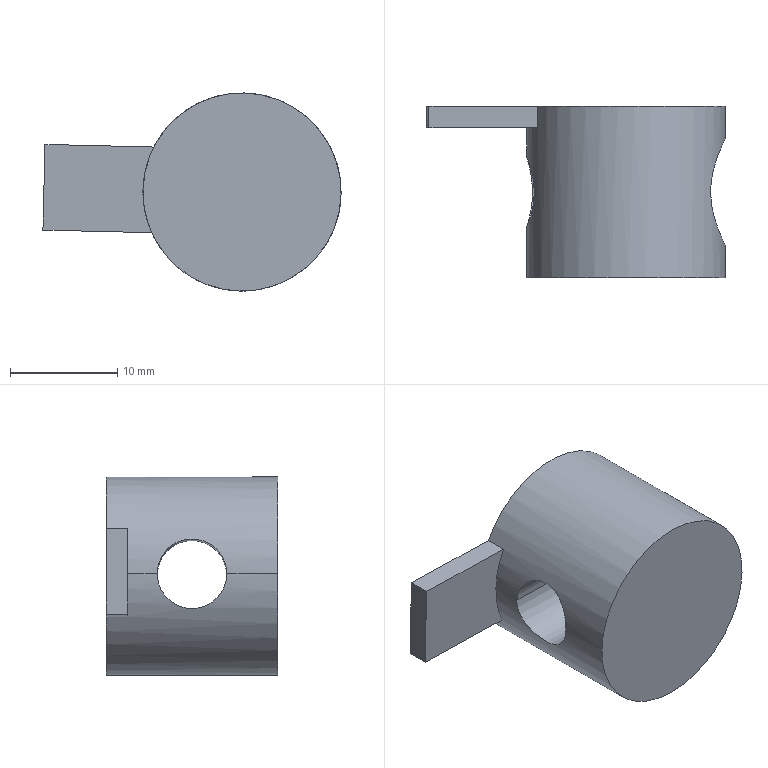Component | SolidWorks | 2012MB0201-1_AUpperRackFrameModule-1_ADJ42-G408-D6.5Assembly-10_Built-inConnectorADJ42-G408-D6.5-1 | 1 solid | 13 faces | box 27.84 x 16 x 18.5 mm | volume 3328 mm3 | plane 7 | cylinder 6 | commonest cylinder face diameters 10 x2 6.5 x2 18.5 x2 | material S45C
build123d program:
from build123d import *

# Parameters (mm, degrees)
SKETCH1_W                                     = 16
SKETCH1_H                                     = 9.25
COUNTERBORE_FOR_M6_HEX_HEAD_BOLT1_D           = 6.5
COUNTERBORE_FOR_M6_HEX_HEAD_BOLT1_CBORE_D     = 10
COUNTERBORE_FOR_M6_HEX_HEAD_BOLT1_CBORE_DEPTH = 12
BOSS_EXTRUDE1_REACH                           = 35.341
BOSS_EXTRUDE1_END_RADIUS                      = 9.25
SKETCH4_W                                     = 2
SKETCH4_H                                     = 8


with BuildPart() as part:
    # Sketch1 → Revolve1 (revolve)
    with BuildSketch(Plane.XY.offset(-18.5), mode=Mode.PRIVATE) as revolve1_sk:
        with Locations((8, 4.625)):
            Rectangle(SKETCH1_W, SKETCH1_H)
    revolve(revolve1_sk.sketch.rotate(Axis((0, 0, -18.5), (1, 0, 0)), 270), axis=Axis((0, 0, -18.5), (1, 0, 0)))

    # Counterbore for M6 Hex Head Bolt1 (through all)
    with Locations(Plane(origin=(8, 0, -27.75), x_dir=(-1, 0, 0), z_dir=(0, 0, -1))):
        with Locations((0, 0)):
            CounterBoreHole(COUNTERBORE_FOR_M6_HEX_HEAD_BOLT1_D / 2, COUNTERBORE_FOR_M6_HEX_HEAD_BOLT1_CBORE_D / 2, COUNTERBORE_FOR_M6_HEX_HEAD_BOLT1_CBORE_DEPTH)

    # Boss-Extrude1: up to this cylinder (the profile starts outside it)
    boss_extrude1_end = Plane(origin=(1, 0, -18.5), z_dir=(1, 0, 0)) * Cylinder(BOSS_EXTRUDE1_END_RADIUS, 90.182, mode=Mode.PRIVATE)
    # Sketch4 → Boss-Extrude1 (add, up to the surface)
    with BuildSketch(Plane.XY, mode=Mode.PRIVATE) as boss_extrude1_sk1:
        with Locations((1, 0)):
            Rectangle(SKETCH4_W, SKETCH4_H)
    boss_extrude1_tool1 = extrude(boss_extrude1_sk1.sketch, amount=-BOSS_EXTRUDE1_REACH, mode=Mode.PRIVATE) - boss_extrude1_end
    add(boss_extrude1_tool1.solids().sort_by_distance((1, 0, 0))[0])


solid = part.part

# Placed as in the assembly
solid = solid.moved(Location((-1764.43, 1041.85, -1140.078), (-0.007146, -88.631, -90.007)))
STEP:
#1=COLOUR_RGB('',0.7922,0.8196,0.9333);
#2=FILL_AREA_STYLE_COLOUR('',#1);
#3=FILL_AREA_STYLE('',(#2));
#4=SURFACE_STYLE_FILL_AREA(#3);
#5=SURFACE_SIDE_STYLE('',(#4));
#6=SURFACE_STYLE_USAGE(.BOTH.,#5);
#7=PRESENTATION_STYLE_ASSIGNMENT((#6));
#8=CARTESIAN_POINT('',(-68.846,40.506,-44.9));
#9=VERTEX_POINT('',#8);
#10=CARTESIAN_POINT('',(-68.846,40.9,-44.9));
#11=VERTEX_POINT('',#10);
#12=CARTESIAN_POINT('',(-68.846,40.703,-44.9));
#13=DIRECTION('',(0.9997,0.,-0.02392));
#14=DIRECTION('',(0.,1.,0.));
#15=AXIS2_PLACEMENT_3D('',#12,#13,#14);
#16=CIRCLE('',#15,0.1969);
#17=EDGE_CURVE('',#9,#11,#16,.T.);
#18=ORIENTED_EDGE('',*,*,#17,.F.);
#19=CARTESIAN_POINT('',(-68.374,40.506,-44.911));
#20=VERTEX_POINT('',#19);
#21=CARTESIAN_POINT('',(-68.374,40.506,-44.911));
#22=DIRECTION('',(0.9997,0.,-0.02392));
#23=VECTOR('',#22,39.37);
#24=LINE('',#21,#23);
#25=EDGE_CURVE('',#9,#20,#24,.T.);
#26=ORIENTED_EDGE('',*,*,#25,.T.);
#27=CARTESIAN_POINT('',(-68.374,40.9,-44.911));
#28=VERTEX_POINT('',#27);
#29=CARTESIAN_POINT('',(-68.374,40.506,-44.911));
#30=CARTESIAN_POINT('',(-68.374,40.506,-44.924));
#31=CARTESIAN_POINT('',(-68.375,40.507,-44.937));
#32=CARTESIAN_POINT('',(-68.378,40.512,-44.963));
#33=CARTESIAN_POINT('',(-68.381,40.516,-44.975));
#34=CARTESIAN_POINT('',(-68.386,40.526,-44.999));
#35=CARTESIAN_POINT('',(-68.39,40.532,-45.01));
#36=CARTESIAN_POINT('',(-68.397,40.547,-45.031));
#37=CARTESIAN_POINT('',(-68.401,40.555,-45.041));
#38=CARTESIAN_POINT('',(-68.409,40.573,-45.059));
#39=CARTESIAN_POINT('',(-68.412,40.582,-45.066));
#40=CARTESIAN_POINT('',(-68.42,40.604,-45.08));
#41=CARTESIAN_POINT('',(-68.423,40.615,-45.086));
#42=CARTESIAN_POINT('',(-68.429,40.638,-45.096));
#43=CARTESIAN_POINT('',(-68.432,40.651,-45.1));
#44=CARTESIAN_POINT('',(-68.435,40.676,-45.105));
#45=CARTESIAN_POINT('',(-68.436,40.689,-45.106));
#46=CARTESIAN_POINT('',(-68.436,40.716,-45.106));
#47=CARTESIAN_POINT('',(-68.435,40.729,-45.105));
#48=CARTESIAN_POINT('',(-68.432,40.754,-45.1));
#49=CARTESIAN_POINT('',(-68.429,40.767,-45.096));
#50=CARTESIAN_POINT('',(-68.423,40.791,-45.087));
#51=CARTESIAN_POINT('',(-68.42,40.802,-45.081));
#52=CARTESIAN_POINT('',(-68.412,40.823,-45.067));
#53=CARTESIAN_POINT('',(-68.409,40.833,-45.059));
#54=CARTESIAN_POINT('',(-68.401,40.851,-45.041));
#55=CARTESIAN_POINT('',(-68.397,40.859,-45.031));
#56=CARTESIAN_POINT('',(-68.391,40.869,-45.016));
#57=CARTESIAN_POINT('',(-68.39,40.873,-45.01));
#58=CARTESIAN_POINT('',(-68.386,40.879,-44.999));
#59=CARTESIAN_POINT('',(-68.385,40.882,-44.993));
#60=CARTESIAN_POINT('',(-68.381,40.889,-44.976));
#61=CARTESIAN_POINT('',(-68.378,40.893,-44.963));
#62=CARTESIAN_POINT('',(-68.375,40.898,-44.938));
#63=CARTESIAN_POINT('',(-68.374,40.9,-44.924));
#64=CARTESIAN_POINT('',(-68.374,40.9,-44.911));
#65=B_SPLINE_CURVE_WITH_KNOTS('',3,(#29,#30,#31,#32,#33,#34,#35,#36,#37,#38,#39,#40,#41,#42,#43,#44,#45,#46,#47,#48,#49,#50,#51,#52,#53,#54,#55,#56,#57,#58,#59,#60,#61,#62,#63,#64),.UNSPECIFIED.,.F.,.F.,(4,2,2,2,2,2,2,2,2,2,2,2,2,2,2,2,2,4),(0.01596,0.01695,0.01795,0.01894,0.01994,0.02093,0.02193,0.02292,0.02392,0.02491,0.02591,0.0269,0.0279,0.02889,0.02939,0.02989,0.03088,0.03188),.UNSPECIFIED.);
#66=EDGE_CURVE('',#20,#28,#65,.T.);
#67=ORIENTED_EDGE('',*,*,#66,.T.);
#68=CARTESIAN_POINT('',(-68.374,40.9,-44.911));
#69=DIRECTION('',(0.9997,0.,-0.02392));
#70=VECTOR('',#69,39.37);
#71=LINE('',#68,#70);
#72=EDGE_CURVE('',#11,#28,#71,.T.);
#73=ORIENTED_EDGE('',*,*,#72,.F.);
#74=EDGE_LOOP('',(#18,#26,#67,#73));
#75=FACE_OUTER_BOUND('',#74,.T.);
#76=CARTESIAN_POINT('',(-68.374,40.703,-44.911));
#77=DIRECTION('',(0.9997,0.,-0.02392));
#78=DIRECTION('',(0.,1.,0.));
#79=AXIS2_PLACEMENT_3D('',#76,#77,#78);
#80=CYLINDRICAL_SURFACE('',#79,0.1969);
#81=ADVANCED_FACE('',(#75),#80,.F.);
#82=CARTESIAN_POINT('',(-69.102,40.831,-44.894));
#83=VERTEX_POINT('',#82);
#84=CARTESIAN_POINT('',(-69.102,40.575,-44.894));
#85=VERTEX_POINT('',#84);
#86=CARTESIAN_POINT('',(-69.102,40.831,-44.894));
#87=CARTESIAN_POINT('',(-69.102,40.831,-44.902));
#88=CARTESIAN_POINT('',(-69.102,40.83,-44.911));
#89=CARTESIAN_POINT('',(-69.101,40.827,-44.927));
#90=CARTESIAN_POINT('',(-69.1,40.824,-44.935));
#91=CARTESIAN_POINT('',(-69.099,40.818,-44.951));
#92=CARTESIAN_POINT('',(-69.098,40.814,-44.958));
#93=CARTESIAN_POINT('',(-69.095,40.804,-44.972));
#94=CARTESIAN_POINT('',(-69.094,40.799,-44.979));
#95=CARTESIAN_POINT('',(-69.09,40.781,-44.996));
#96=CARTESIAN_POINT('',(-69.087,40.767,-45.006));
#97=CARTESIAN_POINT('',(-69.084,40.744,-45.015));
#98=CARTESIAN_POINT('',(-69.083,40.736,-45.018));
#99=CARTESIAN_POINT('',(-69.082,40.72,-45.021));
#100=CARTESIAN_POINT('',(-69.082,40.711,-45.022));
#101=CARTESIAN_POINT('',(-69.082,40.694,-45.022));
#102=CARTESIAN_POINT('',(-69.082,40.686,-45.021));
#103=CARTESIAN_POINT('',(-69.083,40.669,-45.018));
#104=CARTESIAN_POINT('',(-69.084,40.661,-45.015));
#105=CARTESIAN_POINT('',(-69.086,40.646,-45.009));
#106=CARTESIAN_POINT('',(-69.087,40.638,-45.005));
#107=CARTESIAN_POINT('',(-69.09,40.625,-44.996));
#108=CARTESIAN_POINT('',(-69.091,40.618,-44.99));
#109=CARTESIAN_POINT('',(-69.094,40.606,-44.978));
#110=CARTESIAN_POINT('',(-69.095,40.601,-44.972));
#111=CARTESIAN_POINT('',(-69.098,40.592,-44.958));
#112=CARTESIAN_POINT('',(-69.099,40.588,-44.951));
#113=CARTESIAN_POINT('',(-69.1,40.581,-44.935));
#114=CARTESIAN_POINT('',(-69.101,40.579,-44.927));
#115=CARTESIAN_POINT('',(-69.102,40.576,-44.911));
#116=CARTESIAN_POINT('',(-69.102,40.575,-44.902));
#117=CARTESIAN_POINT('',(-69.102,40.575,-44.894));
#118=B_SPLINE_CURVE_WITH_KNOTS('',3,(#86,#87,#88,#89,#90,#91,#92,#93,#94,#95,#96,#97,#98,#99,#100,#101,#102,#103,#104,#105,#106,#107,#108,#109,#110,#111,#112,#113,#114,#115,#116,#117),.UNSPECIFIED.,.F.,.F.,(4,2,2,2,2,2,2,2,2,2,2,2,2,2,2,4),(0.,0.0006402,0.00128,0.001921,0.002561,0.003841,0.004481,0.005122,0.005762,0.006402,0.007042,0.007683,0.008323,0.008963,0.009603,0.01024),.UNSPECIFIED.);
#119=EDGE_CURVE('',#83,#85,#118,.T.);
#120=ORIENTED_EDGE('',*,*,#119,.T.);
#121=CARTESIAN_POINT('',(-68.846,40.575,-44.9));
#122=VERTEX_POINT('',#121);
#123=CARTESIAN_POINT('',(-68.374,40.575,-44.911));
#124=DIRECTION('',(0.9997,0.,-0.02392));
#125=VECTOR('',#124,39.37);
#126=LINE('',#123,#125);
#127=EDGE_CURVE('',#85,#122,#126,.T.);
#128=ORIENTED_EDGE('',*,*,#127,.T.);
#129=CARTESIAN_POINT('',(-68.846,40.831,-44.9));
#130=VERTEX_POINT('',#129);
#131=CARTESIAN_POINT('',(-68.846,40.703,-44.9));
#132=DIRECTION('',(0.9997,0.,-0.02392));
#133=DIRECTION('',(0.,1.,0.));
#134=AXIS2_PLACEMENT_3D('',#131,#132,#133);
#135=CIRCLE('',#134,0.128);
#136=EDGE_CURVE('',#122,#130,#135,.T.);
#137=ORIENTED_EDGE('',*,*,#136,.T.);
#138=CARTESIAN_POINT('',(-68.374,40.831,-44.911));
#139=DIRECTION('',(0.9997,0.,-0.02392));
#140=VECTOR('',#139,39.37);
#141=LINE('',#138,#140);
#142=EDGE_CURVE('',#83,#130,#141,.T.);
#143=ORIENTED_EDGE('',*,*,#142,.F.);
#144=EDGE_LOOP('',(#120,#128,#137,#143));
#145=FACE_OUTER_BOUND('',#144,.T.);
#146=CARTESIAN_POINT('',(-68.374,40.703,-44.911));
#147=DIRECTION('',(0.9997,0.,-0.02392));
#148=DIRECTION('',(0.,1.,0.));
#149=AXIS2_PLACEMENT_3D('',#146,#147,#148);
#150=CYLINDRICAL_SURFACE('',#149,0.128);
#151=ADVANCED_FACE('',(#145),#150,.F.);
#152=CARTESIAN_POINT('',(-69.062,40.939,-44.737));
#153=VERTEX_POINT('',#152);
#154=CARTESIAN_POINT('',(-69.102,40.939,-44.894));
#155=VERTEX_POINT('',#154);
#156=CARTESIAN_POINT('',(-68.738,40.939,-44.902));
#157=DIRECTION('',(0.,-1.,-0.));
#158=DIRECTION('',(0.9997,0.,-0.02392));
#159=AXIS2_PLACEMENT_3D('',#156,#157,#158);
#160=CIRCLE('',#159,0.3642);
#161=EDGE_CURVE('',#153,#155,#160,.T.);
#162=ORIENTED_EDGE('',*,*,#161,.T.);
#163=CARTESIAN_POINT('',(-69.102,41.018,-44.894));
#164=DIRECTION('',(0.,-1.,-0.));
#165=VECTOR('',#164,39.37);
#166=LINE('',#163,#165);
#167=EDGE_CURVE('',#155,#83,#166,.T.);
#168=ORIENTED_EDGE('',*,*,#167,.T.);
#169=CARTESIAN_POINT('',(-69.102,40.575,-44.894));
#170=CARTESIAN_POINT('',(-69.101,40.575,-44.885));
#171=CARTESIAN_POINT('',(-69.101,40.576,-44.877));
#172=CARTESIAN_POINT('',(-69.099,40.579,-44.86));
#173=CARTESIAN_POINT('',(-69.098,40.581,-44.852));
#174=CARTESIAN_POINT('',(-69.096,40.588,-44.837));
#175=CARTESIAN_POINT('',(-69.094,40.592,-44.829));
#176=CARTESIAN_POINT('',(-69.091,40.601,-44.816));
#177=CARTESIAN_POINT('',(-69.09,40.606,-44.809));
#178=CARTESIAN_POINT('',(-69.086,40.618,-44.798));
#179=CARTESIAN_POINT('',(-69.085,40.625,-44.792));
#180=CARTESIAN_POINT('',(-69.082,40.638,-44.783));
#181=CARTESIAN_POINT('',(-69.08,40.646,-44.779));
#182=CARTESIAN_POINT('',(-69.078,40.661,-44.773));
#183=CARTESIAN_POINT('',(-69.077,40.669,-44.77));
#184=CARTESIAN_POINT('',(-69.076,40.686,-44.767));
#185=CARTESIAN_POINT('',(-69.075,40.694,-44.766));
#186=CARTESIAN_POINT('',(-69.075,40.711,-44.766));
#187=CARTESIAN_POINT('',(-69.076,40.72,-44.767));
#188=CARTESIAN_POINT('',(-69.077,40.736,-44.77));
#189=CARTESIAN_POINT('',(-69.078,40.744,-44.773));
#190=CARTESIAN_POINT('',(-69.08,40.76,-44.779));
#191=CARTESIAN_POINT('',(-69.082,40.767,-44.783));
#192=CARTESIAN_POINT('',(-69.085,40.781,-44.792));
#193=CARTESIAN_POINT('',(-69.086,40.787,-44.798));
#194=CARTESIAN_POINT('',(-69.09,40.799,-44.809));
#195=CARTESIAN_POINT('',(-69.091,40.804,-44.816));
#196=CARTESIAN_POINT('',(-69.094,40.814,-44.83));
#197=CARTESIAN_POINT('',(-69.096,40.818,-44.837));
#198=CARTESIAN_POINT('',(-69.098,40.824,-44.852));
#199=CARTESIAN_POINT('',(-69.099,40.827,-44.86));
#200=CARTESIAN_POINT('',(-69.101,40.83,-44.877));
#201=CARTESIAN_POINT('',(-69.101,40.831,-44.885));
#202=CARTESIAN_POINT('',(-69.102,40.831,-44.894));
#203=B_SPLINE_CURVE_WITH_KNOTS('',3,(#169,#170,#171,#172,#173,#174,#175,#176,#177,#178,#179,#180,#181,#182,#183,#184,#185,#186,#187,#188,#189,#190,#191,#192,#193,#194,#195,#196,#197,#198,#199,#200,#201,#202),.UNSPECIFIED.,.F.,.F.,(4,2,2,2,2,2,2,2,2,2,2,2,2,2,2,2,4),(0.01024,0.01088,0.01152,0.01216,0.0128,0.01344,0.01408,0.01472,0.01536,0.016,0.01664,0.01728,0.01792,0.01856,0.0192,0.01984,0.02048),.UNSPECIFIED.);
#204=EDGE_CURVE('',#85,#83,#203,.T.);
#205=ORIENTED_EDGE('',*,*,#204,.F.);
#206=CARTESIAN_POINT('',(-69.102,40.388,-44.894));
#207=VERTEX_POINT('',#206);
#208=CARTESIAN_POINT('',(-69.102,41.018,-44.894));
#209=DIRECTION('',(0.,-1.,-0.));
#210=VECTOR('',#209,39.37);
#211=LINE('',#208,#210);
#212=EDGE_CURVE('',#85,#207,#211,.T.);
#213=ORIENTED_EDGE('',*,*,#212,.T.);
#214=CARTESIAN_POINT('',(-68.374,40.388,-44.911));
#215=VERTEX_POINT('',#214);
#216=CARTESIAN_POINT('',(-68.738,40.388,-44.902));
#217=DIRECTION('',(0.,-1.,-0.));
#218=DIRECTION('',(0.9997,0.,-0.02392));
#219=AXIS2_PLACEMENT_3D('',#216,#217,#218);
#220=CIRCLE('',#219,0.3642);
#221=EDGE_CURVE('',#215,#207,#220,.T.);
#222=ORIENTED_EDGE('',*,*,#221,.F.);
#223=CARTESIAN_POINT('',(-68.374,41.018,-44.911));
#224=DIRECTION('',(0.,-1.,-0.));
#225=VECTOR('',#224,39.37);
#226=LINE('',#223,#225);
#227=EDGE_CURVE('',#20,#215,#226,.T.);
#228=ORIENTED_EDGE('',*,*,#227,.F.);
#229=CARTESIAN_POINT('',(-68.374,40.9,-44.911));
#230=CARTESIAN_POINT('',(-68.373,40.9,-44.898));
#231=CARTESIAN_POINT('',(-68.374,40.898,-44.885));
#232=CARTESIAN_POINT('',(-68.376,40.893,-44.859));
#233=CARTESIAN_POINT('',(-68.378,40.889,-44.846));
#234=CARTESIAN_POINT('',(-68.382,40.879,-44.823));
#235=CARTESIAN_POINT('',(-68.385,40.873,-44.811));
#236=CARTESIAN_POINT('',(-68.391,40.859,-44.79));
#237=CARTESIAN_POINT('',(-68.394,40.851,-44.78));
#238=CARTESIAN_POINT('',(-68.401,40.833,-44.762));
#239=CARTESIAN_POINT('',(-68.405,40.823,-44.754));
#240=CARTESIAN_POINT('',(-68.412,40.802,-44.74));
#241=CARTESIAN_POINT('',(-68.415,40.791,-44.733));
#242=CARTESIAN_POINT('',(-68.42,40.767,-44.723));
#243=CARTESIAN_POINT('',(-68.423,40.755,-44.719));
#244=CARTESIAN_POINT('',(-68.426,40.729,-44.714));
#245=CARTESIAN_POINT('',(-68.427,40.716,-44.713));
#246=CARTESIAN_POINT('',(-68.427,40.696,-44.713));
#247=CARTESIAN_POINT('',(-68.426,40.69,-44.713));
#248=CARTESIAN_POINT('',(-68.426,40.677,-44.715));
#249=CARTESIAN_POINT('',(-68.425,40.67,-44.716));
#250=CARTESIAN_POINT('',(-68.423,40.657,-44.718));
#251=CARTESIAN_POINT('',(-68.423,40.651,-44.72));
#252=CARTESIAN_POINT('',(-68.42,40.639,-44.724));
#253=CARTESIAN_POINT('',(-68.419,40.633,-44.726));
#254=CARTESIAN_POINT('',(-68.415,40.615,-44.733));
#255=CARTESIAN_POINT('',(-68.412,40.604,-44.74));
#256=CARTESIAN_POINT('',(-68.405,40.582,-44.754));
#257=CARTESIAN_POINT('',(-68.401,40.573,-44.762));
#258=CARTESIAN_POINT('',(-68.394,40.555,-44.78));
#259=CARTESIAN_POINT('',(-68.391,40.547,-44.79));
#260=CARTESIAN_POINT('',(-68.385,40.532,-44.811));
#261=CARTESIAN_POINT('',(-68.382,40.526,-44.823));
#262=CARTESIAN_POINT('',(-68.379,40.519,-44.841));
#263=CARTESIAN_POINT('',(-68.378,40.517,-44.847));
#264=CARTESIAN_POINT('',(-68.376,40.513,-44.859));
#265=CARTESIAN_POINT('',(-68.375,40.511,-44.866));
#266=CARTESIAN_POINT('',(-68.374,40.507,-44.885));
#267=CARTESIAN_POINT('',(-68.373,40.506,-44.898));
#268=CARTESIAN_POINT('',(-68.374,40.506,-44.911));
#269=B_SPLINE_CURVE_WITH_KNOTS('',3,(#229,#230,#231,#232,#233,#234,#235,#236,#237,#238,#239,#240,#241,#242,#243,#244,#245,#246,#247,#248,#249,#250,#251,#252,#253,#254,#255,#256,#257,#258,#259,#260,#261,#262,#263,#264,#265,#266,#267,#268),.UNSPECIFIED.,.F.,.F.,(4,2,2,2,2,2,2,2,2,2,2,2,2,2,2,2,2,2,2,4),(0.,0.0009973,0.001995,0.002992,0.003989,0.004987,0.005984,0.006981,0.007979,0.008477,0.008976,0.009475,0.009973,0.01097,0.01197,0.01297,0.01396,0.01446,0.01496,0.01596),.UNSPECIFIED.);
#270=EDGE_CURVE('',#28,#20,#269,.T.);
#271=ORIENTED_EDGE('',*,*,#270,.F.);
#272=CARTESIAN_POINT('',(-68.374,41.018,-44.911));
#273=VERTEX_POINT('',#272);
#274=CARTESIAN_POINT('',(-68.374,41.018,-44.911));
#275=DIRECTION('',(0.,-1.,-0.));
#276=VECTOR('',#275,39.37);
#277=LINE('',#274,#276);
#278=EDGE_CURVE('',#273,#28,#277,.T.);
#279=ORIENTED_EDGE('',*,*,#278,.F.);
#280=CARTESIAN_POINT('',(-69.062,41.018,-44.737));
#281=VERTEX_POINT('',#280);
#282=CARTESIAN_POINT('',(-68.738,41.018,-44.902));
#283=DIRECTION('',(0.,-1.,-0.));
#284=DIRECTION('',(0.9997,0.,-0.02392));
#285=AXIS2_PLACEMENT_3D('',#282,#283,#284);
#286=CIRCLE('',#285,0.3642);
#287=EDGE_CURVE('',#273,#281,#286,.T.);
#288=ORIENTED_EDGE('',*,*,#287,.T.);
#289=CARTESIAN_POINT('',(-69.062,41.018,-44.737));
#290=DIRECTION('',(0.,-1.,-0.));
#291=VECTOR('',#290,39.37);
#292=LINE('',#289,#291);
#293=EDGE_CURVE('',#281,#153,#292,.T.);
#294=ORIENTED_EDGE('',*,*,#293,.T.);
#295=EDGE_LOOP('',(#162,#168,#205,#213,#222,#228,#271,#279,#288,#294));
#296=FACE_OUTER_BOUND('',#295,.T.);
#297=CARTESIAN_POINT('',(-68.738,41.018,-44.902));
#298=DIRECTION('',(0.,-1.,-0.));
#299=DIRECTION('',(0.9997,0.,-0.02392));
#300=AXIS2_PLACEMENT_3D('',#297,#298,#299);
#301=CYLINDRICAL_SURFACE('',#300,0.3642);
#302=ADVANCED_FACE('',(#296),#301,.T.);
#303=ORIENTED_EDGE('',*,*,#167,.F.);
#304=CARTESIAN_POINT('',(-69.07,40.939,-45.052));
#305=VERTEX_POINT('',#304);
#306=CARTESIAN_POINT('',(-68.738,40.939,-44.902));
#307=DIRECTION('',(0.,-1.,-0.));
#308=DIRECTION('',(0.9997,0.,-0.02392));
#309=AXIS2_PLACEMENT_3D('',#306,#307,#308);
#310=CIRCLE('',#309,0.3642);
#311=EDGE_CURVE('',#155,#305,#310,.T.);
#312=ORIENTED_EDGE('',*,*,#311,.T.);
#313=CARTESIAN_POINT('',(-69.07,41.018,-45.052));
#314=VERTEX_POINT('',#313);
#315=CARTESIAN_POINT('',(-69.07,41.018,-45.052));
#316=DIRECTION('',(-0.,1.,0.));
#317=VECTOR('',#316,39.37);
#318=LINE('',#315,#317);
#319=EDGE_CURVE('',#305,#314,#318,.T.);
#320=ORIENTED_EDGE('',*,*,#319,.T.);
#321=CARTESIAN_POINT('',(-68.738,41.018,-44.902));
#322=DIRECTION('',(0.,-1.,-0.));
#323=DIRECTION('',(0.9997,0.,-0.02392));
#324=AXIS2_PLACEMENT_3D('',#321,#322,#323);
#325=CIRCLE('',#324,0.3642);
#326=EDGE_CURVE('',#314,#273,#325,.T.);
#327=ORIENTED_EDGE('',*,*,#326,.T.);
#328=ORIENTED_EDGE('',*,*,#278,.T.);
#329=ORIENTED_EDGE('',*,*,#66,.F.);
#330=ORIENTED_EDGE('',*,*,#227,.T.);
#331=CARTESIAN_POINT('',(-68.738,40.388,-44.902));
#332=DIRECTION('',(0.,-1.,-0.));
#333=DIRECTION('',(0.9997,0.,-0.02392));
#334=AXIS2_PLACEMENT_3D('',#331,#332,#333);
#335=CIRCLE('',#334,0.3642);
#336=EDGE_CURVE('',#207,#215,#335,.T.);
#337=ORIENTED_EDGE('',*,*,#336,.F.);
#338=ORIENTED_EDGE('',*,*,#212,.F.);
#339=ORIENTED_EDGE('',*,*,#119,.F.);
#340=EDGE_LOOP('',(#303,#312,#320,#327,#328,#329,#330,#337,#338,#339));
#341=FACE_OUTER_BOUND('',#340,.T.);
#342=CARTESIAN_POINT('',(-68.738,41.018,-44.902));
#343=DIRECTION('',(0.,-1.,-0.));
#344=DIRECTION('',(0.9997,0.,-0.02392));
#345=AXIS2_PLACEMENT_3D('',#342,#343,#344);
#346=CYLINDRICAL_SURFACE('',#345,0.3642);
#347=ADVANCED_FACE('',(#341),#346,.T.);
#348=ORIENTED_EDGE('',*,*,#326,.F.);
#349=CARTESIAN_POINT('',(-69.47,41.018,-45.042));
#350=VERTEX_POINT('',#349);
#351=CARTESIAN_POINT('',(-68.377,41.018,-45.068));
#352=DIRECTION('',(-0.9997,-0.,0.02392));
#353=VECTOR('',#352,39.37);
#354=LINE('',#351,#353);
#355=EDGE_CURVE('',#314,#350,#354,.T.);
#356=ORIENTED_EDGE('',*,*,#355,.T.);
#357=CARTESIAN_POINT('',(-69.462,41.018,-44.727));
#358=VERTEX_POINT('',#357);
#359=CARTESIAN_POINT('',(-69.462,41.018,-44.727));
#360=DIRECTION('',(-0.02392,0.,-0.9997));
#361=VECTOR('',#360,39.37);
#362=LINE('',#359,#361);
#363=EDGE_CURVE('',#358,#350,#362,.T.);
#364=ORIENTED_EDGE('',*,*,#363,.F.);
#365=CARTESIAN_POINT('',(-68.37,41.018,-44.754));
#366=DIRECTION('',(-0.9997,-0.,0.02392));
#367=VECTOR('',#366,39.37);
#368=LINE('',#365,#367);
#369=EDGE_CURVE('',#281,#358,#368,.T.);
#370=ORIENTED_EDGE('',*,*,#369,.F.);
#371=ORIENTED_EDGE('',*,*,#287,.F.);
#372=EDGE_LOOP('',(#348,#356,#364,#370,#371));
#373=FACE_OUTER_BOUND('',#372,.T.);
#374=CARTESIAN_POINT('',(-68.729,41.018,-44.538));
#375=DIRECTION('',(-0.,1.,0.));
#376=DIRECTION('',(-0.9997,-0.,0.02392));
#377=AXIS2_PLACEMENT_3D('',#374,#375,#376);
#378=PLANE('',#377);
#379=ADVANCED_FACE('',(#373),#378,.T.);
#380=ORIENTED_EDGE('',*,*,#221,.T.);
#381=ORIENTED_EDGE('',*,*,#336,.T.);
#382=EDGE_LOOP('',(#380,#381));
#383=FACE_OUTER_BOUND('',#382,.T.);
#384=CARTESIAN_POINT('',(-68.738,40.388,-44.902));
#385=DIRECTION('',(0.,-1.,-0.));
#386=DIRECTION('',(0.9997,0.,-0.02392));
#387=AXIS2_PLACEMENT_3D('',#384,#385,#386);
#388=PLANE('',#387);
#389=ADVANCED_FACE('',(#383),#388,.T.);
#390=ORIENTED_EDGE('',*,*,#127,.F.);
#391=ORIENTED_EDGE('',*,*,#204,.T.);
#392=ORIENTED_EDGE('',*,*,#142,.T.);
#393=CARTESIAN_POINT('',(-68.846,40.703,-44.9));
#394=DIRECTION('',(0.9997,0.,-0.02392));
#395=DIRECTION('',(0.,1.,0.));
#396=AXIS2_PLACEMENT_3D('',#393,#394,#395);
#397=CIRCLE('',#396,0.128);
#398=EDGE_CURVE('',#130,#122,#397,.T.);
#399=ORIENTED_EDGE('',*,*,#398,.T.);
#400=EDGE_LOOP('',(#390,#391,#392,#399));
#401=FACE_OUTER_BOUND('',#400,.T.);
#402=CARTESIAN_POINT('',(-68.374,40.703,-44.911));
#403=DIRECTION('',(0.9997,0.,-0.02392));
#404=DIRECTION('',(0.,1.,0.));
#405=AXIS2_PLACEMENT_3D('',#402,#403,#404);
#406=CYLINDRICAL_SURFACE('',#405,0.128);
#407=ADVANCED_FACE('',(#401),#406,.F.);
#408=ORIENTED_EDGE('',*,*,#398,.F.);
#409=ORIENTED_EDGE('',*,*,#136,.F.);
#410=EDGE_LOOP('',(#408,#409));
#411=FACE_BOUND('',#410,.T.);
#412=CARTESIAN_POINT('',(-68.846,40.703,-44.9));
#413=DIRECTION('',(0.9997,0.,-0.02392));
#414=DIRECTION('',(0.,1.,0.));
#415=AXIS2_PLACEMENT_3D('',#412,#413,#414);
#416=CIRCLE('',#415,0.1969);
#417=EDGE_CURVE('',#11,#9,#416,.T.);
#418=ORIENTED_EDGE('',*,*,#417,.T.);
#419=ORIENTED_EDGE('',*,*,#17,.T.);
#420=EDGE_LOOP('',(#418,#419));
#421=FACE_OUTER_BOUND('',#420,.T.);
#422=CARTESIAN_POINT('',(-68.846,40.575,-44.9));
#423=DIRECTION('',(-0.9997,-0.,0.02392));
#424=DIRECTION('',(0.,-1.,-0.));
#425=AXIS2_PLACEMENT_3D('',#422,#423,#424);
#426=PLANE('',#425);
#427=ADVANCED_FACE('',(#411,#421),#426,.F.);
#428=ORIENTED_EDGE('',*,*,#25,.F.);
#429=ORIENTED_EDGE('',*,*,#417,.F.);
#430=ORIENTED_EDGE('',*,*,#72,.T.);
#431=ORIENTED_EDGE('',*,*,#270,.T.);
#432=EDGE_LOOP('',(#428,#429,#430,#431));
#433=FACE_OUTER_BOUND('',#432,.T.);
#434=CARTESIAN_POINT('',(-68.374,40.703,-44.911));
#435=DIRECTION('',(0.9997,0.,-0.02392));
#436=DIRECTION('',(0.,1.,0.));
#437=AXIS2_PLACEMENT_3D('',#434,#435,#436);
#438=CYLINDRICAL_SURFACE('',#437,0.1969);
#439=ADVANCED_FACE('',(#433),#438,.F.);
#440=ORIENTED_EDGE('',*,*,#293,.F.);
#441=ORIENTED_EDGE('',*,*,#369,.T.);
#442=CARTESIAN_POINT('',(-69.462,40.939,-44.727));
#443=VERTEX_POINT('',#442);
#444=CARTESIAN_POINT('',(-69.462,40.939,-44.727));
#445=DIRECTION('',(-0.,1.,0.));
#446=VECTOR('',#445,39.37);
#447=LINE('',#444,#446);
#448=EDGE_CURVE('',#443,#358,#447,.T.);
#449=ORIENTED_EDGE('',*,*,#448,.F.);
#450=CARTESIAN_POINT('',(-68.37,40.939,-44.754));
#451=DIRECTION('',(-0.9997,-0.,0.02392));
#452=VECTOR('',#451,39.37);
#453=LINE('',#450,#452);
#454=EDGE_CURVE('',#153,#443,#453,.T.);
#455=ORIENTED_EDGE('',*,*,#454,.F.);
#456=EDGE_LOOP('',(#440,#441,#449,#455));
#457=FACE_OUTER_BOUND('',#456,.T.);
#458=CARTESIAN_POINT('',(-68.37,40.939,-44.754));
#459=DIRECTION('',(0.02392,-0.,0.9997));
#460=DIRECTION('',(-0.9997,-0.,0.02392));
#461=AXIS2_PLACEMENT_3D('',#458,#459,#460);
#462=PLANE('',#461);
#463=ADVANCED_FACE('',(#457),#462,.T.);
#464=ORIENTED_EDGE('',*,*,#363,.T.);
#465=CARTESIAN_POINT('',(-69.47,40.939,-45.042));
#466=VERTEX_POINT('',#465);
#467=CARTESIAN_POINT('',(-69.47,41.018,-45.042));
#468=DIRECTION('',(0.,-1.,-0.));
#469=VECTOR('',#468,39.37);
#470=LINE('',#467,#469);
#471=EDGE_CURVE('',#350,#466,#470,.T.);
#472=ORIENTED_EDGE('',*,*,#471,.T.);
#473=CARTESIAN_POINT('',(-69.47,40.939,-45.042));
#474=DIRECTION('',(0.02392,-0.,0.9997));
#475=VECTOR('',#474,39.37);
#476=LINE('',#473,#475);
#477=EDGE_CURVE('',#466,#443,#476,.T.);
#478=ORIENTED_EDGE('',*,*,#477,.T.);
#479=ORIENTED_EDGE('',*,*,#448,.T.);
#480=EDGE_LOOP('',(#464,#472,#478,#479));
#481=FACE_OUTER_BOUND('',#480,.T.);
#482=CARTESIAN_POINT('',(-69.466,41.018,-44.885));
#483=DIRECTION('',(-0.9997,-0.,0.02392));
#484=DIRECTION('',(0.,-1.,-0.));
#485=AXIS2_PLACEMENT_3D('',#482,#483,#484);
#486=PLANE('',#485);
#487=ADVANCED_FACE('',(#481),#486,.T.);
#488=ORIENTED_EDGE('',*,*,#161,.F.);
#489=ORIENTED_EDGE('',*,*,#454,.T.);
#490=ORIENTED_EDGE('',*,*,#477,.F.);
#491=CARTESIAN_POINT('',(-68.377,40.939,-45.068));
#492=DIRECTION('',(-0.9997,-0.,0.02392));
#493=VECTOR('',#492,39.37);
#494=LINE('',#491,#493);
#495=EDGE_CURVE('',#305,#466,#494,.T.);
#496=ORIENTED_EDGE('',*,*,#495,.F.);
#497=ORIENTED_EDGE('',*,*,#311,.F.);
#498=EDGE_LOOP('',(#488,#489,#490,#496,#497));
#499=FACE_OUTER_BOUND('',#498,.T.);
#500=CARTESIAN_POINT('',(-68.377,40.939,-45.068));
#501=DIRECTION('',(0.,-1.,-0.));
#502=DIRECTION('',(0.9997,0.,-0.02392));
#503=AXIS2_PLACEMENT_3D('',#500,#501,#502);
#504=PLANE('',#503);
#505=ADVANCED_FACE('',(#499),#504,.T.);
#506=ORIENTED_EDGE('',*,*,#319,.F.);
#507=ORIENTED_EDGE('',*,*,#495,.T.);
#508=ORIENTED_EDGE('',*,*,#471,.F.);
#509=ORIENTED_EDGE('',*,*,#355,.F.);
#510=EDGE_LOOP('',(#506,#507,#508,#509));
#511=FACE_OUTER_BOUND('',#510,.T.);
#512=CARTESIAN_POINT('',(-68.377,41.018,-45.068));
#513=DIRECTION('',(-0.02392,0.,-0.9997));
#514=DIRECTION('',(0.9997,0.,-0.02392));
#515=AXIS2_PLACEMENT_3D('',#512,#513,#514);
#516=PLANE('',#515);
#517=ADVANCED_FACE('',(#511),#516,.T.);
#518=CLOSED_SHELL('',(#81,#151,#302,#347,#379,#389,#407,#427,#439,#463,#487,#505,#517));
#519=MANIFOLD_SOLID_BREP('',#518);
#520=STYLED_ITEM('',(#7),#519);
#521=(LENGTH_UNIT()NAMED_UNIT(*)SI_UNIT($,.METRE.));
#522=LENGTH_MEASURE_WITH_UNIT(LENGTH_MEASURE(0.0254),#521);
#523=DIMENSIONAL_EXPONENTS(1.,0.,0.,0.,0.,0.,0.);
#524=(CONVERSION_BASED_UNIT('',#522)LENGTH_UNIT()NAMED_UNIT(#523));
#525=UNCERTAINTY_MEASURE_WITH_UNIT(LENGTH_MEASURE(0.00001),#524,'','');
#526=(NAMED_UNIT(*)PLANE_ANGLE_UNIT()SI_UNIT($,.RADIAN.));
#527=(NAMED_UNIT(*)SI_UNIT($,.STERADIAN.)SOLID_ANGLE_UNIT());
#528=(GEOMETRIC_REPRESENTATION_CONTEXT(3)GLOBAL_UNCERTAINTY_ASSIGNED_CONTEXT((#525))GLOBAL_UNIT_ASSIGNED_CONTEXT((#524,#526,#527))REPRESENTATION_CONTEXT('',''));
#529=MECHANICAL_DESIGN_GEOMETRIC_PRESENTATION_REPRESENTATION('',(#520),#528);
#530=CARTESIAN_POINT('',(0.,0.,0.));
#531=DIRECTION('',(0.,0.,1.));
#532=DIRECTION('',(1.,0.,0.));
#533=AXIS2_PLACEMENT_3D('',#530,#531,#532);
#534=(LENGTH_UNIT()NAMED_UNIT(*)SI_UNIT($,.METRE.));
#535=LENGTH_MEASURE_WITH_UNIT(LENGTH_MEASURE(0.0254),#534);
#536=DIMENSIONAL_EXPONENTS(1.,0.,0.,0.,0.,0.,0.);
#537=(CONVERSION_BASED_UNIT('',#535)LENGTH_UNIT()NAMED_UNIT(#536));
#538=UNCERTAINTY_MEASURE_WITH_UNIT(LENGTH_MEASURE(0.00001),#537,'','');
#539=(NAMED_UNIT(*)PLANE_ANGLE_UNIT()SI_UNIT($,.RADIAN.));
#540=(NAMED_UNIT(*)SI_UNIT($,.STERADIAN.)SOLID_ANGLE_UNIT());
#541=(GEOMETRIC_REPRESENTATION_CONTEXT(3)GLOBAL_UNCERTAINTY_ASSIGNED_CONTEXT((#538))GLOBAL_UNIT_ASSIGNED_CONTEXT((#537,#539,#540))REPRESENTATION_CONTEXT('',''));
#542=ADVANCED_BREP_SHAPE_REPRESENTATION('',(#519,#533),#541);
#543=PRESENTATION_LAYER_ASSIGNMENT('','',(#520));